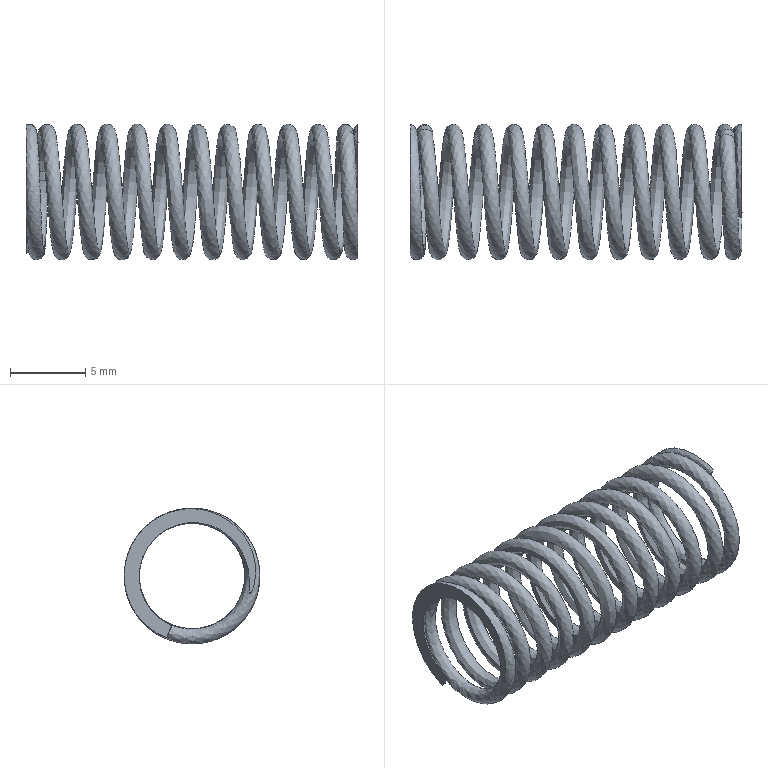Component | NX | SPRING_CYLINDER_COMPRESSION_1_2 | 1 solid | 9 faces | volume 239 mm3 | spline 5 | plane 4